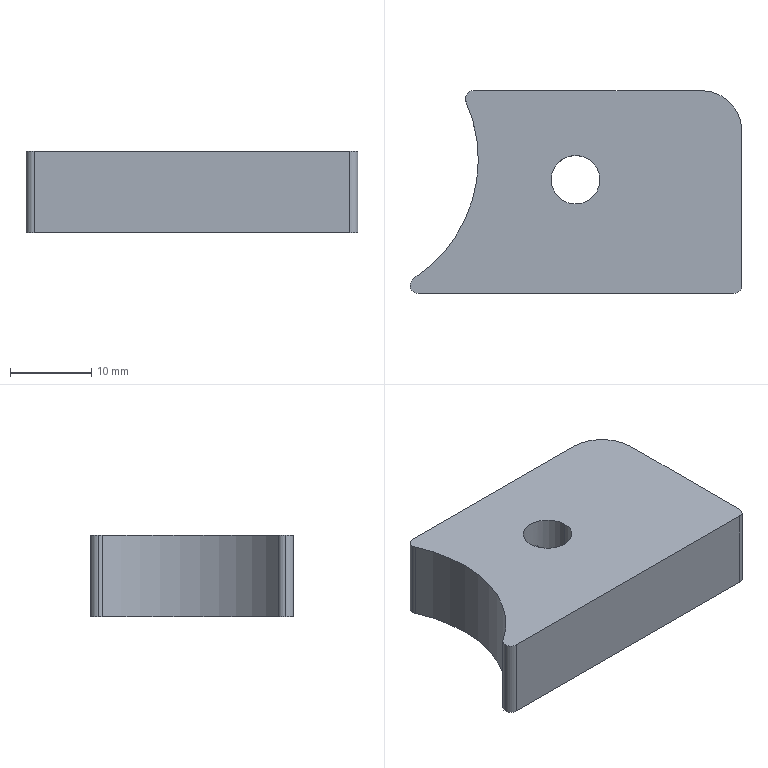Component | SolidWorks | Assembly5.1-1_Part1.1-2 | 1 solid | 16 faces | box 40.9 x 25 x 10 mm | volume 8268 mm3 | cylinder 11 | plane 5 | commonest cylinder face diameters 2 x5 3.3 x2 6 x2 35 x1 10 x1
build123d program:
from build123d import *

# Parameters (mm, degrees)
SKETCH1_R             = 3
BOSS_EXTRUDE1_DEPTH   = 10
M4_TAPPED_HOLE1_D     = 3.3
M4_TAPPED_HOLE1_DEPTH = 12
M4_TAPPED_HOLE1_TIP   = 0.9914


with BuildPart() as part:
    # Sketch1 → Boss-Extrude1 (new body)
    with BuildSketch(Plane.XY):
        with BuildLine():
            Line((2.1, 0), (41, 0))
            ThreePointArc((41, 0), (41.707, 0.2929), (42, 1))
            Line((42, 1), (42, 20))
            ThreePointArc((42, 20), (40.536, 23.536), (37, 25))
            Line((37, 25), (8.912, 25))
            ThreePointArc((8.912, 25), (8.073, 24.545), (7.997, 23.595))
            ThreePointArc((7.997, 23.595), (8.78, 11.53), (1.554, 1.838))
            ThreePointArc((1.554, 1.838), (1.141, 0.7153), (2.1, 0))
        make_face()
        with Locations((21.5, 14)):
            Circle(SKETCH1_R, mode=Mode.SUBTRACT)
    extrude(amount=BOSS_EXTRUDE1_DEPTH)

    # M4 Tapped Hole1
    with Locations(Plane(origin=(0, 25, 0), x_dir=(1, 0, 0), z_dir=(0, 1, 0))):
        with Locations((21.5, -5)):
            Hole(M4_TAPPED_HOLE1_D / 2, depth=M4_TAPPED_HOLE1_DEPTH)
            with Locations((0, 0, -(M4_TAPPED_HOLE1_DEPTH + M4_TAPPED_HOLE1_TIP / 2))):  # 118° drill point
                Cone(0, M4_TAPPED_HOLE1_D / 2, M4_TAPPED_HOLE1_TIP, mode=Mode.SUBTRACT)


solid = part.part

# Placed as in the assembly
solid = solid.moved(Location((48.5, 150, -19.741), (0, 0, 0)))
STEP:
#1=COLOUR_RGB('',0.7922,0.8196,0.9333);
#2=FILL_AREA_STYLE_COLOUR('',#1);
#3=FILL_AREA_STYLE('',(#2));
#4=SURFACE_STYLE_FILL_AREA(#3);
#5=SURFACE_SIDE_STYLE('',(#4));
#6=SURFACE_STYLE_USAGE(.BOTH.,#5);
#7=PRESENTATION_STYLE_ASSIGNMENT((#6));
#8=CARTESIAN_POINT('',(2.756,6.575,-0.5154));
#9=VERTEX_POINT('',#8);
#10=CARTESIAN_POINT('',(2.756,6.575,-0.6453));
#11=VERTEX_POINT('',#10);
#12=CARTESIAN_POINT('',(2.756,6.575,-0.5154));
#13=CARTESIAN_POINT('',(2.752,6.575,-0.5154));
#14=CARTESIAN_POINT('',(2.747,6.575,-0.5158));
#15=CARTESIAN_POINT('',(2.739,6.574,-0.5175));
#16=CARTESIAN_POINT('',(2.735,6.573,-0.5188));
#17=CARTESIAN_POINT('',(2.723,6.57,-0.5238));
#18=CARTESIAN_POINT('',(2.716,6.568,-0.5286));
#19=CARTESIAN_POINT('',(2.704,6.563,-0.5404));
#20=CARTESIAN_POINT('',(2.699,6.56,-0.5474));
#21=CARTESIAN_POINT('',(2.694,6.558,-0.5591));
#22=CARTESIAN_POINT('',(2.693,6.557,-0.5632));
#23=CARTESIAN_POINT('',(2.691,6.556,-0.5716));
#24=CARTESIAN_POINT('',(2.691,6.555,-0.5759));
#25=CARTESIAN_POINT('',(2.691,6.555,-0.5846));
#26=CARTESIAN_POINT('',(2.691,6.556,-0.589));
#27=CARTESIAN_POINT('',(2.693,6.557,-0.5974));
#28=CARTESIAN_POINT('',(2.694,6.558,-0.6016));
#29=CARTESIAN_POINT('',(2.699,6.56,-0.6133));
#30=CARTESIAN_POINT('',(2.704,6.563,-0.6204));
#31=CARTESIAN_POINT('',(2.716,6.568,-0.6321));
#32=CARTESIAN_POINT('',(2.723,6.57,-0.637));
#33=CARTESIAN_POINT('',(2.735,6.573,-0.6419));
#34=CARTESIAN_POINT('',(2.739,6.574,-0.6432));
#35=CARTESIAN_POINT('',(2.747,6.575,-0.6449));
#36=CARTESIAN_POINT('',(2.752,6.575,-0.6453));
#37=CARTESIAN_POINT('',(2.756,6.575,-0.6453));
#38=B_SPLINE_CURVE_WITH_KNOTS('',3,(#12,#13,#14,#15,#16,#17,#18,#19,#20,#21,#22,#23,#24,#25,#26,#27,#28,#29,#30,#31,#32,#33,#34,#35,#36,#37),.UNSPECIFIED.,.F.,.F.,(4,2,2,2,2,2,2,2,2,2,2,2,4),(0.,0.0003294,0.0006588,0.001318,0.001976,0.002306,0.002635,0.002965,0.003294,0.003953,0.004612,0.004941,0.00527),.UNSPECIFIED.);
#39=EDGE_CURVE('',#9,#11,#38,.T.);
#40=ORIENTED_EDGE('',*,*,#39,.T.);
#41=CARTESIAN_POINT('',(2.756,6.89,-0.6453));
#42=VERTEX_POINT('',#41);
#43=CARTESIAN_POINT('',(2.756,6.89,-0.6453));
#44=DIRECTION('',(0.,1.,0.));
#45=VECTOR('',#44,39.37);
#46=LINE('',#43,#45);
#47=EDGE_CURVE('',#11,#42,#46,.T.);
#48=ORIENTED_EDGE('',*,*,#47,.T.);
#49=CARTESIAN_POINT('',(2.756,6.89,-0.5154));
#50=VERTEX_POINT('',#49);
#51=CARTESIAN_POINT('',(2.756,6.89,-0.5804));
#52=DIRECTION('',(0.,1.,0.));
#53=DIRECTION('',(0.,0.,1.));
#54=AXIS2_PLACEMENT_3D('',#51,#52,#53);
#55=CIRCLE('',#54,0.06496);
#56=EDGE_CURVE('',#42,#50,#55,.T.);
#57=ORIENTED_EDGE('',*,*,#56,.T.);
#58=CARTESIAN_POINT('',(2.756,6.89,-0.5154));
#59=DIRECTION('',(0.,1.,0.));
#60=VECTOR('',#59,39.37);
#61=LINE('',#58,#60);
#62=EDGE_CURVE('',#9,#50,#61,.T.);
#63=ORIENTED_EDGE('',*,*,#62,.F.);
#64=EDGE_LOOP('',(#40,#48,#57,#63));
#65=FACE_OUTER_BOUND('',#64,.T.);
#66=CARTESIAN_POINT('',(2.756,6.89,-0.5804));
#67=DIRECTION('',(0.,1.,0.));
#68=DIRECTION('',(0.,0.,1.));
#69=AXIS2_PLACEMENT_3D('',#66,#67,#68);
#70=CYLINDRICAL_SURFACE('',#69,0.06496);
#71=ADVANCED_FACE('',(#65),#70,.F.);
#72=CARTESIAN_POINT('',(2.638,6.457,-0.3835));
#73=VERTEX_POINT('',#72);
#74=CARTESIAN_POINT('',(2.874,6.457,-0.3835));
#75=VERTEX_POINT('',#74);
#76=CARTESIAN_POINT('',(2.756,6.457,-0.3835));
#77=DIRECTION('',(0.,0.,1.));
#78=DIRECTION('',(1.,0.,0.));
#79=AXIS2_PLACEMENT_3D('',#76,#77,#78);
#80=CIRCLE('',#79,0.1181);
#81=EDGE_CURVE('',#73,#75,#80,.T.);
#82=ORIENTED_EDGE('',*,*,#81,.T.);
#83=CARTESIAN_POINT('',(2.874,6.457,-0.7772));
#84=VERTEX_POINT('',#83);
#85=CARTESIAN_POINT('',(2.874,6.457,-0.3835));
#86=DIRECTION('',(0.,0.,-1.));
#87=VECTOR('',#86,39.37);
#88=LINE('',#85,#87);
#89=EDGE_CURVE('',#75,#84,#88,.T.);
#90=ORIENTED_EDGE('',*,*,#89,.T.);
#91=CARTESIAN_POINT('',(2.638,6.457,-0.7772));
#92=VERTEX_POINT('',#91);
#93=CARTESIAN_POINT('',(2.756,6.457,-0.7772));
#94=DIRECTION('',(0.,0.,1.));
#95=DIRECTION('',(1.,0.,0.));
#96=AXIS2_PLACEMENT_3D('',#93,#94,#95);
#97=CIRCLE('',#96,0.1181);
#98=EDGE_CURVE('',#92,#84,#97,.T.);
#99=ORIENTED_EDGE('',*,*,#98,.F.);
#100=CARTESIAN_POINT('',(2.638,6.457,-0.3835));
#101=DIRECTION('',(0.,0.,-1.));
#102=VECTOR('',#101,39.37);
#103=LINE('',#100,#102);
#104=EDGE_CURVE('',#73,#92,#103,.T.);
#105=ORIENTED_EDGE('',*,*,#104,.F.);
#106=EDGE_LOOP('',(#82,#90,#99,#105));
#107=FACE_OUTER_BOUND('',#106,.T.);
#108=CARTESIAN_POINT('',(2.756,6.457,-0.3835));
#109=DIRECTION('',(0.,0.,-1.));
#110=DIRECTION('',(-1.,0.,0.));
#111=AXIS2_PLACEMENT_3D('',#108,#109,#110);
#112=CYLINDRICAL_SURFACE('',#111,0.1181);
#113=ADVANCED_FACE('',(#107),#112,.F.);
#114=CARTESIAN_POINT('',(1.953,5.945,-0.3835));
#115=VERTEX_POINT('',#114);
#116=CARTESIAN_POINT('',(1.992,5.906,-0.3835));
#117=VERTEX_POINT('',#116);
#118=CARTESIAN_POINT('',(1.992,5.945,-0.3835));
#119=DIRECTION('',(0.,0.,1.));
#120=DIRECTION('',(-1.,0.,0.));
#121=AXIS2_PLACEMENT_3D('',#118,#119,#120);
#122=CIRCLE('',#121,0.03937);
#123=EDGE_CURVE('',#115,#117,#122,.T.);
#124=ORIENTED_EDGE('',*,*,#123,.F.);
#125=CARTESIAN_POINT('',(1.953,5.945,-0.7772));
#126=VERTEX_POINT('',#125);
#127=CARTESIAN_POINT('',(1.953,5.945,-0.3835));
#128=DIRECTION('',(0.,0.,-1.));
#129=VECTOR('',#128,39.37);
#130=LINE('',#127,#129);
#131=EDGE_CURVE('',#115,#126,#130,.T.);
#132=ORIENTED_EDGE('',*,*,#131,.T.);
#133=CARTESIAN_POINT('',(1.992,5.906,-0.7772));
#134=VERTEX_POINT('',#133);
#135=CARTESIAN_POINT('',(1.992,5.945,-0.7772));
#136=DIRECTION('',(0.,0.,1.));
#137=DIRECTION('',(-1.,0.,0.));
#138=AXIS2_PLACEMENT_3D('',#135,#136,#137);
#139=CIRCLE('',#138,0.03937);
#140=EDGE_CURVE('',#126,#134,#139,.T.);
#141=ORIENTED_EDGE('',*,*,#140,.T.);
#142=CARTESIAN_POINT('',(1.992,5.906,-0.3835));
#143=DIRECTION('',(0.,0.,-1.));
#144=VECTOR('',#143,39.37);
#145=LINE('',#142,#144);
#146=EDGE_CURVE('',#117,#134,#145,.T.);
#147=ORIENTED_EDGE('',*,*,#146,.F.);
#148=EDGE_LOOP('',(#124,#132,#141,#147));
#149=FACE_OUTER_BOUND('',#148,.T.);
#150=CARTESIAN_POINT('',(1.992,5.945,-0.3835));
#151=DIRECTION('',(0.,0.,-1.));
#152=DIRECTION('',(-1.,0.,0.));
#153=AXIS2_PLACEMENT_3D('',#150,#151,#152);
#154=CYLINDRICAL_SURFACE('',#153,0.03937);
#155=ADVANCED_FACE('',(#149),#154,.T.);
#156=CARTESIAN_POINT('',(2.221,6.85,-0.3835));
#157=VERTEX_POINT('',#156);
#158=CARTESIAN_POINT('',(2.224,6.834,-0.3835));
#159=VERTEX_POINT('',#158);
#160=CARTESIAN_POINT('',(2.26,6.85,-0.3835));
#161=DIRECTION('',(0.,0.,1.));
#162=DIRECTION('',(-1.,0.,0.));
#163=AXIS2_PLACEMENT_3D('',#160,#161,#162);
#164=CIRCLE('',#163,0.03937);
#165=EDGE_CURVE('',#157,#159,#164,.T.);
#166=ORIENTED_EDGE('',*,*,#165,.F.);
#167=CARTESIAN_POINT('',(2.221,6.85,-0.7772));
#168=VERTEX_POINT('',#167);
#169=CARTESIAN_POINT('',(2.221,6.85,-0.3835));
#170=DIRECTION('',(0.,0.,-1.));
#171=VECTOR('',#170,39.37);
#172=LINE('',#169,#171);
#173=EDGE_CURVE('',#157,#168,#172,.T.);
#174=ORIENTED_EDGE('',*,*,#173,.T.);
#175=CARTESIAN_POINT('',(2.224,6.834,-0.7772));
#176=VERTEX_POINT('',#175);
#177=CARTESIAN_POINT('',(2.26,6.85,-0.7772));
#178=DIRECTION('',(0.,0.,1.));
#179=DIRECTION('',(-1.,0.,0.));
#180=AXIS2_PLACEMENT_3D('',#177,#178,#179);
#181=CIRCLE('',#180,0.03937);
#182=EDGE_CURVE('',#168,#176,#181,.T.);
#183=ORIENTED_EDGE('',*,*,#182,.T.);
#184=CARTESIAN_POINT('',(2.224,6.834,-0.3835));
#185=DIRECTION('',(0.,0.,-1.));
#186=VECTOR('',#185,39.37);
#187=LINE('',#184,#186);
#188=EDGE_CURVE('',#159,#176,#187,.T.);
#189=ORIENTED_EDGE('',*,*,#188,.F.);
#190=EDGE_LOOP('',(#166,#174,#183,#189));
#191=FACE_OUTER_BOUND('',#190,.T.);
#192=CARTESIAN_POINT('',(2.26,6.85,-0.3835));
#193=DIRECTION('',(0.,0.,-1.));
#194=DIRECTION('',(-1.,0.,0.));
#195=AXIS2_PLACEMENT_3D('',#192,#193,#194);
#196=CYLINDRICAL_SURFACE('',#195,0.03937);
#197=ADVANCED_FACE('',(#191),#196,.T.);
#198=CARTESIAN_POINT('',(2.26,6.89,-0.3835));
#199=VERTEX_POINT('',#198);
#200=CARTESIAN_POINT('',(2.26,6.85,-0.3835));
#201=DIRECTION('',(0.,0.,1.));
#202=DIRECTION('',(-1.,0.,0.));
#203=AXIS2_PLACEMENT_3D('',#200,#201,#202);
#204=CIRCLE('',#203,0.03937);
#205=EDGE_CURVE('',#199,#157,#204,.T.);
#206=ORIENTED_EDGE('',*,*,#205,.T.);
#207=ORIENTED_EDGE('',*,*,#165,.T.);
#208=CARTESIAN_POINT('',(1.971,5.978,-0.3835));
#209=VERTEX_POINT('',#208);
#210=CARTESIAN_POINT('',(1.594,6.555,-0.3835));
#211=DIRECTION('',(0.,0.,-1.));
#212=DIRECTION('',(1.,0.,0.));
#213=AXIS2_PLACEMENT_3D('',#210,#211,#212);
#214=CIRCLE('',#213,0.689);
#215=EDGE_CURVE('',#159,#209,#214,.T.);
#216=ORIENTED_EDGE('',*,*,#215,.T.);
#217=CARTESIAN_POINT('',(1.992,5.945,-0.3835));
#218=DIRECTION('',(0.,0.,1.));
#219=DIRECTION('',(-1.,0.,0.));
#220=AXIS2_PLACEMENT_3D('',#217,#218,#219);
#221=CIRCLE('',#220,0.03937);
#222=EDGE_CURVE('',#209,#115,#221,.T.);
#223=ORIENTED_EDGE('',*,*,#222,.T.);
#224=ORIENTED_EDGE('',*,*,#123,.T.);
#225=CARTESIAN_POINT('',(3.524,5.906,-0.3835));
#226=VERTEX_POINT('',#225);
#227=CARTESIAN_POINT('',(1.992,5.906,-0.3835));
#228=DIRECTION('',(1.,-0.,0.));
#229=VECTOR('',#228,39.37);
#230=LINE('',#227,#229);
#231=EDGE_CURVE('',#117,#226,#230,.T.);
#232=ORIENTED_EDGE('',*,*,#231,.T.);
#233=CARTESIAN_POINT('',(3.563,5.945,-0.3835));
#234=VERTEX_POINT('',#233);
#235=CARTESIAN_POINT('',(3.524,5.945,-0.3835));
#236=DIRECTION('',(0.,0.,1.));
#237=DIRECTION('',(1.,0.,0.));
#238=AXIS2_PLACEMENT_3D('',#235,#236,#237);
#239=CIRCLE('',#238,0.03937);
#240=EDGE_CURVE('',#226,#234,#239,.T.);
#241=ORIENTED_EDGE('',*,*,#240,.T.);
#242=CARTESIAN_POINT('',(3.563,6.693,-0.3835));
#243=VERTEX_POINT('',#242);
#244=CARTESIAN_POINT('',(3.563,5.945,-0.3835));
#245=DIRECTION('',(0.,1.,0.));
#246=VECTOR('',#245,39.37);
#247=LINE('',#244,#246);
#248=EDGE_CURVE('',#234,#243,#247,.T.);
#249=ORIENTED_EDGE('',*,*,#248,.T.);
#250=CARTESIAN_POINT('',(3.366,6.89,-0.3835));
#251=VERTEX_POINT('',#250);
#252=CARTESIAN_POINT('',(3.366,6.693,-0.3835));
#253=DIRECTION('',(0.,0.,1.));
#254=DIRECTION('',(1.,0.,0.));
#255=AXIS2_PLACEMENT_3D('',#252,#253,#254);
#256=CIRCLE('',#255,0.1969);
#257=EDGE_CURVE('',#243,#251,#256,.T.);
#258=ORIENTED_EDGE('',*,*,#257,.T.);
#259=CARTESIAN_POINT('',(3.366,6.89,-0.3835));
#260=DIRECTION('',(-1.,0.,0.));
#261=VECTOR('',#260,39.37);
#262=LINE('',#259,#261);
#263=EDGE_CURVE('',#251,#199,#262,.T.);
#264=ORIENTED_EDGE('',*,*,#263,.T.);
#265=EDGE_LOOP('',(#206,#207,#216,#223,#224,#232,#241,#249,#258,#264));
#266=FACE_OUTER_BOUND('',#265,.T.);
#267=ORIENTED_EDGE('',*,*,#81,.F.);
#268=CARTESIAN_POINT('',(2.756,6.457,-0.3835));
#269=DIRECTION('',(0.,0.,1.));
#270=DIRECTION('',(1.,0.,0.));
#271=AXIS2_PLACEMENT_3D('',#268,#269,#270);
#272=CIRCLE('',#271,0.1181);
#273=EDGE_CURVE('',#75,#73,#272,.T.);
#274=ORIENTED_EDGE('',*,*,#273,.F.);
#275=EDGE_LOOP('',(#267,#274));
#276=FACE_BOUND('',#275,.T.);
#277=CARTESIAN_POINT('',(2.26,6.85,-0.3835));
#278=DIRECTION('',(0.,0.,-1.));
#279=DIRECTION('',(-1.,0.,0.));
#280=AXIS2_PLACEMENT_3D('',#277,#278,#279);
#281=PLANE('',#280);
#282=ADVANCED_FACE('',(#266,#276),#281,.F.);
#283=CARTESIAN_POINT('',(2.26,6.89,-0.7772));
#284=VERTEX_POINT('',#283);
#285=CARTESIAN_POINT('',(2.26,6.85,-0.7772));
#286=DIRECTION('',(0.,0.,1.));
#287=DIRECTION('',(-1.,0.,0.));
#288=AXIS2_PLACEMENT_3D('',#285,#286,#287);
#289=CIRCLE('',#288,0.03937);
#290=EDGE_CURVE('',#284,#168,#289,.T.);
#291=ORIENTED_EDGE('',*,*,#290,.F.);
#292=CARTESIAN_POINT('',(3.366,6.89,-0.7772));
#293=VERTEX_POINT('',#292);
#294=CARTESIAN_POINT('',(3.366,6.89,-0.7772));
#295=DIRECTION('',(-1.,0.,0.));
#296=VECTOR('',#295,39.37);
#297=LINE('',#294,#296);
#298=EDGE_CURVE('',#293,#284,#297,.T.);
#299=ORIENTED_EDGE('',*,*,#298,.F.);
#300=CARTESIAN_POINT('',(3.563,6.693,-0.7772));
#301=VERTEX_POINT('',#300);
#302=CARTESIAN_POINT('',(3.366,6.693,-0.7772));
#303=DIRECTION('',(0.,0.,1.));
#304=DIRECTION('',(1.,0.,0.));
#305=AXIS2_PLACEMENT_3D('',#302,#303,#304);
#306=CIRCLE('',#305,0.1969);
#307=EDGE_CURVE('',#301,#293,#306,.T.);
#308=ORIENTED_EDGE('',*,*,#307,.F.);
#309=CARTESIAN_POINT('',(3.563,5.945,-0.7772));
#310=VERTEX_POINT('',#309);
#311=CARTESIAN_POINT('',(3.563,5.945,-0.7772));
#312=DIRECTION('',(0.,1.,0.));
#313=VECTOR('',#312,39.37);
#314=LINE('',#311,#313);
#315=EDGE_CURVE('',#310,#301,#314,.T.);
#316=ORIENTED_EDGE('',*,*,#315,.F.);
#317=CARTESIAN_POINT('',(3.524,5.906,-0.7772));
#318=VERTEX_POINT('',#317);
#319=CARTESIAN_POINT('',(3.524,5.945,-0.7772));
#320=DIRECTION('',(0.,0.,1.));
#321=DIRECTION('',(1.,0.,0.));
#322=AXIS2_PLACEMENT_3D('',#319,#320,#321);
#323=CIRCLE('',#322,0.03937);
#324=EDGE_CURVE('',#318,#310,#323,.T.);
#325=ORIENTED_EDGE('',*,*,#324,.F.);
#326=CARTESIAN_POINT('',(1.992,5.906,-0.7772));
#327=DIRECTION('',(1.,-0.,0.));
#328=VECTOR('',#327,39.37);
#329=LINE('',#326,#328);
#330=EDGE_CURVE('',#134,#318,#329,.T.);
#331=ORIENTED_EDGE('',*,*,#330,.F.);
#332=ORIENTED_EDGE('',*,*,#140,.F.);
#333=CARTESIAN_POINT('',(1.971,5.978,-0.7772));
#334=VERTEX_POINT('',#333);
#335=CARTESIAN_POINT('',(1.992,5.945,-0.7772));
#336=DIRECTION('',(0.,0.,1.));
#337=DIRECTION('',(-1.,0.,0.));
#338=AXIS2_PLACEMENT_3D('',#335,#336,#337);
#339=CIRCLE('',#338,0.03937);
#340=EDGE_CURVE('',#334,#126,#339,.T.);
#341=ORIENTED_EDGE('',*,*,#340,.F.);
#342=CARTESIAN_POINT('',(1.594,6.555,-0.7772));
#343=DIRECTION('',(0.,0.,-1.));
#344=DIRECTION('',(1.,0.,0.));
#345=AXIS2_PLACEMENT_3D('',#342,#343,#344);
#346=CIRCLE('',#345,0.689);
#347=EDGE_CURVE('',#176,#334,#346,.T.);
#348=ORIENTED_EDGE('',*,*,#347,.F.);
#349=ORIENTED_EDGE('',*,*,#182,.F.);
#350=EDGE_LOOP('',(#291,#299,#308,#316,#325,#331,#332,#341,#348,#349));
#351=FACE_OUTER_BOUND('',#350,.T.);
#352=ORIENTED_EDGE('',*,*,#98,.T.);
#353=CARTESIAN_POINT('',(2.756,6.457,-0.7772));
#354=DIRECTION('',(0.,0.,1.));
#355=DIRECTION('',(1.,0.,0.));
#356=AXIS2_PLACEMENT_3D('',#353,#354,#355);
#357=CIRCLE('',#356,0.1181);
#358=EDGE_CURVE('',#84,#92,#357,.T.);
#359=ORIENTED_EDGE('',*,*,#358,.T.);
#360=EDGE_LOOP('',(#352,#359));
#361=FACE_BOUND('',#360,.T.);
#362=CARTESIAN_POINT('',(2.26,6.85,-0.7772));
#363=DIRECTION('',(0.,0.,-1.));
#364=DIRECTION('',(-1.,0.,0.));
#365=AXIS2_PLACEMENT_3D('',#362,#363,#364);
#366=PLANE('',#365);
#367=ADVANCED_FACE('',(#351,#361),#366,.T.);
#368=ORIENTED_EDGE('',*,*,#173,.F.);
#369=ORIENTED_EDGE('',*,*,#205,.F.);
#370=CARTESIAN_POINT('',(2.26,6.89,-0.3835));
#371=DIRECTION('',(0.,0.,-1.));
#372=VECTOR('',#371,39.37);
#373=LINE('',#370,#372);
#374=EDGE_CURVE('',#199,#284,#373,.T.);
#375=ORIENTED_EDGE('',*,*,#374,.T.);
#376=ORIENTED_EDGE('',*,*,#290,.T.);
#377=EDGE_LOOP('',(#368,#369,#375,#376));
#378=FACE_OUTER_BOUND('',#377,.T.);
#379=CARTESIAN_POINT('',(2.26,6.85,-0.3835));
#380=DIRECTION('',(0.,0.,-1.));
#381=DIRECTION('',(-1.,0.,0.));
#382=AXIS2_PLACEMENT_3D('',#379,#380,#381);
#383=CYLINDRICAL_SURFACE('',#382,0.03937);
#384=ADVANCED_FACE('',(#378),#383,.T.);
#385=ORIENTED_EDGE('',*,*,#347,.T.);
#386=CARTESIAN_POINT('',(1.971,5.978,-0.3835));
#387=DIRECTION('',(0.,0.,-1.));
#388=VECTOR('',#387,39.37);
#389=LINE('',#386,#388);
#390=EDGE_CURVE('',#209,#334,#389,.T.);
#391=ORIENTED_EDGE('',*,*,#390,.F.);
#392=ORIENTED_EDGE('',*,*,#215,.F.);
#393=ORIENTED_EDGE('',*,*,#188,.T.);
#394=EDGE_LOOP('',(#385,#391,#392,#393));
#395=FACE_OUTER_BOUND('',#394,.T.);
#396=CARTESIAN_POINT('',(1.594,6.555,-0.3835));
#397=DIRECTION('',(0.,0.,-1.));
#398=DIRECTION('',(-1.,0.,0.));
#399=AXIS2_PLACEMENT_3D('',#396,#397,#398);
#400=CYLINDRICAL_SURFACE('',#399,0.689);
#401=ADVANCED_FACE('',(#395),#400,.F.);
#402=ORIENTED_EDGE('',*,*,#131,.F.);
#403=ORIENTED_EDGE('',*,*,#222,.F.);
#404=ORIENTED_EDGE('',*,*,#390,.T.);
#405=ORIENTED_EDGE('',*,*,#340,.T.);
#406=EDGE_LOOP('',(#402,#403,#404,#405));
#407=FACE_OUTER_BOUND('',#406,.T.);
#408=CARTESIAN_POINT('',(1.992,5.945,-0.3835));
#409=DIRECTION('',(0.,0.,-1.));
#410=DIRECTION('',(-1.,0.,0.));
#411=AXIS2_PLACEMENT_3D('',#408,#409,#410);
#412=CYLINDRICAL_SURFACE('',#411,0.03937);
#413=ADVANCED_FACE('',(#407),#412,.T.);
#414=ORIENTED_EDGE('',*,*,#330,.T.);
#415=CARTESIAN_POINT('',(3.524,5.906,-0.3835));
#416=DIRECTION('',(0.,0.,-1.));
#417=VECTOR('',#416,39.37);
#418=LINE('',#415,#417);
#419=EDGE_CURVE('',#226,#318,#418,.T.);
#420=ORIENTED_EDGE('',*,*,#419,.F.);
#421=ORIENTED_EDGE('',*,*,#231,.F.);
#422=ORIENTED_EDGE('',*,*,#146,.T.);
#423=EDGE_LOOP('',(#414,#420,#421,#422));
#424=FACE_OUTER_BOUND('',#423,.T.);
#425=CARTESIAN_POINT('',(1.992,5.906,-0.3835));
#426=DIRECTION('',(0.,1.,0.));
#427=DIRECTION('',(-1.,0.,0.));
#428=AXIS2_PLACEMENT_3D('',#425,#426,#427);
#429=PLANE('',#428);
#430=ADVANCED_FACE('',(#424),#429,.F.);
#431=ORIENTED_EDGE('',*,*,#324,.T.);
#432=CARTESIAN_POINT('',(3.563,5.945,-0.3835));
#433=DIRECTION('',(0.,0.,-1.));
#434=VECTOR('',#433,39.37);
#435=LINE('',#432,#434);
#436=EDGE_CURVE('',#234,#310,#435,.T.);
#437=ORIENTED_EDGE('',*,*,#436,.F.);
#438=ORIENTED_EDGE('',*,*,#240,.F.);
#439=ORIENTED_EDGE('',*,*,#419,.T.);
#440=EDGE_LOOP('',(#431,#437,#438,#439));
#441=FACE_OUTER_BOUND('',#440,.T.);
#442=CARTESIAN_POINT('',(3.524,5.945,-0.3835));
#443=DIRECTION('',(0.,0.,-1.));
#444=DIRECTION('',(-1.,0.,0.));
#445=AXIS2_PLACEMENT_3D('',#442,#443,#444);
#446=CYLINDRICAL_SURFACE('',#445,0.03937);
#447=ADVANCED_FACE('',(#441),#446,.T.);
#448=ORIENTED_EDGE('',*,*,#315,.T.);
#449=CARTESIAN_POINT('',(3.563,6.693,-0.3835));
#450=DIRECTION('',(0.,0.,-1.));
#451=VECTOR('',#450,39.37);
#452=LINE('',#449,#451);
#453=EDGE_CURVE('',#243,#301,#452,.T.);
#454=ORIENTED_EDGE('',*,*,#453,.F.);
#455=ORIENTED_EDGE('',*,*,#248,.F.);
#456=ORIENTED_EDGE('',*,*,#436,.T.);
#457=EDGE_LOOP('',(#448,#454,#455,#456));
#458=FACE_OUTER_BOUND('',#457,.T.);
#459=CARTESIAN_POINT('',(3.563,5.945,-0.3835));
#460=DIRECTION('',(-1.,0.,0.));
#461=DIRECTION('',(0.,0.,1.));
#462=AXIS2_PLACEMENT_3D('',#459,#460,#461);
#463=PLANE('',#462);
#464=ADVANCED_FACE('',(#458),#463,.F.);
#465=ORIENTED_EDGE('',*,*,#307,.T.);
#466=CARTESIAN_POINT('',(3.366,6.89,-0.3835));
#467=DIRECTION('',(0.,0.,-1.));
#468=VECTOR('',#467,39.37);
#469=LINE('',#466,#468);
#470=EDGE_CURVE('',#251,#293,#469,.T.);
#471=ORIENTED_EDGE('',*,*,#470,.F.);
#472=ORIENTED_EDGE('',*,*,#257,.F.);
#473=ORIENTED_EDGE('',*,*,#453,.T.);
#474=EDGE_LOOP('',(#465,#471,#472,#473));
#475=FACE_OUTER_BOUND('',#474,.T.);
#476=CARTESIAN_POINT('',(3.366,6.693,-0.3835));
#477=DIRECTION('',(0.,0.,-1.));
#478=DIRECTION('',(-1.,0.,0.));
#479=AXIS2_PLACEMENT_3D('',#476,#477,#478);
#480=CYLINDRICAL_SURFACE('',#479,0.1969);
#481=ADVANCED_FACE('',(#475),#480,.T.);
#482=CARTESIAN_POINT('',(2.756,6.89,-0.5804));
#483=DIRECTION('',(0.,1.,0.));
#484=DIRECTION('',(0.,0.,1.));
#485=AXIS2_PLACEMENT_3D('',#482,#483,#484);
#486=CIRCLE('',#485,0.06496);
#487=EDGE_CURVE('',#50,#42,#486,.T.);
#488=ORIENTED_EDGE('',*,*,#487,.F.);
#489=ORIENTED_EDGE('',*,*,#56,.F.);
#490=EDGE_LOOP('',(#488,#489));
#491=FACE_BOUND('',#490,.T.);
#492=ORIENTED_EDGE('',*,*,#298,.T.);
#493=ORIENTED_EDGE('',*,*,#374,.F.);
#494=ORIENTED_EDGE('',*,*,#263,.F.);
#495=ORIENTED_EDGE('',*,*,#470,.T.);
#496=EDGE_LOOP('',(#492,#493,#494,#495));
#497=FACE_OUTER_BOUND('',#496,.T.);
#498=CARTESIAN_POINT('',(3.366,6.89,-0.3835));
#499=DIRECTION('',(-0.,-1.,0.));
#500=DIRECTION('',(1.,-0.,0.));
#501=AXIS2_PLACEMENT_3D('',#498,#499,#500);
#502=PLANE('',#501);
#503=ADVANCED_FACE('',(#491,#497),#502,.F.);
#504=ORIENTED_EDGE('',*,*,#89,.F.);
#505=ORIENTED_EDGE('',*,*,#273,.T.);
#506=ORIENTED_EDGE('',*,*,#104,.T.);
#507=ORIENTED_EDGE('',*,*,#358,.F.);
#508=EDGE_LOOP('',(#504,#505,#506,#507));
#509=FACE_OUTER_BOUND('',#508,.T.);
#510=ORIENTED_EDGE('',*,*,#39,.F.);
#511=CARTESIAN_POINT('',(2.756,6.575,-0.6453));
#512=CARTESIAN_POINT('',(2.76,6.575,-0.6453));
#513=CARTESIAN_POINT('',(2.765,6.575,-0.6449));
#514=CARTESIAN_POINT('',(2.773,6.574,-0.6432));
#515=CARTESIAN_POINT('',(2.777,6.573,-0.6419));
#516=CARTESIAN_POINT('',(2.785,6.571,-0.6386));
#517=CARTESIAN_POINT('',(2.789,6.57,-0.6365));
#518=CARTESIAN_POINT('',(2.796,6.568,-0.6318));
#519=CARTESIAN_POINT('',(2.799,6.567,-0.6291));
#520=CARTESIAN_POINT('',(2.808,6.563,-0.6203));
#521=CARTESIAN_POINT('',(2.813,6.56,-0.6133));
#522=CARTESIAN_POINT('',(2.819,6.557,-0.5978));
#523=CARTESIAN_POINT('',(2.821,6.555,-0.5891));
#524=CARTESIAN_POINT('',(2.821,6.555,-0.5761));
#525=CARTESIAN_POINT('',(2.82,6.556,-0.5717));
#526=CARTESIAN_POINT('',(2.819,6.557,-0.5633));
#527=CARTESIAN_POINT('',(2.817,6.558,-0.5592));
#528=CARTESIAN_POINT('',(2.814,6.559,-0.5513));
#529=CARTESIAN_POINT('',(2.812,6.561,-0.5476));
#530=CARTESIAN_POINT('',(2.808,6.563,-0.5407));
#531=CARTESIAN_POINT('',(2.805,6.564,-0.5374));
#532=CARTESIAN_POINT('',(2.799,6.567,-0.5315));
#533=CARTESIAN_POINT('',(2.796,6.568,-0.5289));
#534=CARTESIAN_POINT('',(2.789,6.57,-0.5242));
#535=CARTESIAN_POINT('',(2.785,6.571,-0.5221));
#536=CARTESIAN_POINT('',(2.773,6.574,-0.5172));
#537=CARTESIAN_POINT('',(2.765,6.575,-0.5154));
#538=CARTESIAN_POINT('',(2.756,6.575,-0.5154));
#539=B_SPLINE_CURVE_WITH_KNOTS('',3,(#511,#512,#513,#514,#515,#516,#517,#518,#519,#520,#521,#522,#523,#524,#525,#526,#527,#528,#529,#530,#531,#532,#533,#534,#535,#536,#537,#538),.UNSPECIFIED.,.F.,.F.,(4,2,2,2,2,2,2,2,2,2,2,2,2,4),(0.00527,0.005599,0.005928,0.006256,0.006585,0.007242,0.007899,0.008228,0.008556,0.008885,0.009213,0.009542,0.009871,0.01053),.UNSPECIFIED.);
#540=EDGE_CURVE('',#11,#9,#539,.T.);
#541=ORIENTED_EDGE('',*,*,#540,.F.);
#542=EDGE_LOOP('',(#510,#541));
#543=FACE_BOUND('',#542,.T.);
#544=CARTESIAN_POINT('',(2.756,6.457,-0.3835));
#545=DIRECTION('',(0.,0.,-1.));
#546=DIRECTION('',(-1.,0.,0.));
#547=AXIS2_PLACEMENT_3D('',#544,#545,#546);
#548=CYLINDRICAL_SURFACE('',#547,0.1181);
#549=ADVANCED_FACE('',(#509,#543),#548,.F.);
#550=ORIENTED_EDGE('',*,*,#47,.F.);
#551=ORIENTED_EDGE('',*,*,#540,.T.);
#552=ORIENTED_EDGE('',*,*,#62,.T.);
#553=ORIENTED_EDGE('',*,*,#487,.T.);
#554=EDGE_LOOP('',(#550,#551,#552,#553));
#555=FACE_OUTER_BOUND('',#554,.T.);
#556=CARTESIAN_POINT('',(2.756,6.89,-0.5804));
#557=DIRECTION('',(0.,1.,0.));
#558=DIRECTION('',(0.,0.,1.));
#559=AXIS2_PLACEMENT_3D('',#556,#557,#558);
#560=CYLINDRICAL_SURFACE('',#559,0.06496);
#561=ADVANCED_FACE('',(#555),#560,.F.);
#562=CLOSED_SHELL('',(#71,#113,#155,#197,#282,#367,#384,#401,#413,#430,#447,#464,#481,#503,#549,#561));
#563=MANIFOLD_SOLID_BREP('',#562);
#564=STYLED_ITEM('',(#7),#563);
#565=(LENGTH_UNIT()NAMED_UNIT(*)SI_UNIT($,.METRE.));
#566=LENGTH_MEASURE_WITH_UNIT(LENGTH_MEASURE(0.0254),#565);
#567=DIMENSIONAL_EXPONENTS(1.,0.,0.,0.,0.,0.,0.);
#568=(CONVERSION_BASED_UNIT('',#566)LENGTH_UNIT()NAMED_UNIT(#567));
#569=UNCERTAINTY_MEASURE_WITH_UNIT(LENGTH_MEASURE(0.00001),#568,'','');
#570=(NAMED_UNIT(*)PLANE_ANGLE_UNIT()SI_UNIT($,.RADIAN.));
#571=(NAMED_UNIT(*)SI_UNIT($,.STERADIAN.)SOLID_ANGLE_UNIT());
#572=(GEOMETRIC_REPRESENTATION_CONTEXT(3)GLOBAL_UNCERTAINTY_ASSIGNED_CONTEXT((#569))GLOBAL_UNIT_ASSIGNED_CONTEXT((#568,#570,#571))REPRESENTATION_CONTEXT('',''));
#573=MECHANICAL_DESIGN_GEOMETRIC_PRESENTATION_REPRESENTATION('',(#564),#572);
#574=PRESENTATION_LAYER_ASSIGNMENT('','',(#564));
#575=CARTESIAN_POINT('',(0.,0.,0.));
#576=DIRECTION('',(0.,0.,1.));
#577=DIRECTION('',(1.,0.,0.));
#578=AXIS2_PLACEMENT_3D('',#575,#576,#577);
#579=(LENGTH_UNIT()NAMED_UNIT(*)SI_UNIT($,.METRE.));
#580=LENGTH_MEASURE_WITH_UNIT(LENGTH_MEASURE(0.0254),#579);
#581=DIMENSIONAL_EXPONENTS(1.,0.,0.,0.,0.,0.,0.);
#582=(CONVERSION_BASED_UNIT('',#580)LENGTH_UNIT()NAMED_UNIT(#581));
#583=UNCERTAINTY_MEASURE_WITH_UNIT(LENGTH_MEASURE(0.00001),#582,'','');
#584=(NAMED_UNIT(*)PLANE_ANGLE_UNIT()SI_UNIT($,.RADIAN.));
#585=(NAMED_UNIT(*)SI_UNIT($,.STERADIAN.)SOLID_ANGLE_UNIT());
#586=(GEOMETRIC_REPRESENTATION_CONTEXT(3)GLOBAL_UNCERTAINTY_ASSIGNED_CONTEXT((#583))GLOBAL_UNIT_ASSIGNED_CONTEXT((#582,#584,#585))REPRESENTATION_CONTEXT('',''));
#587=ADVANCED_BREP_SHAPE_REPRESENTATION('',(#563,#578),#586);